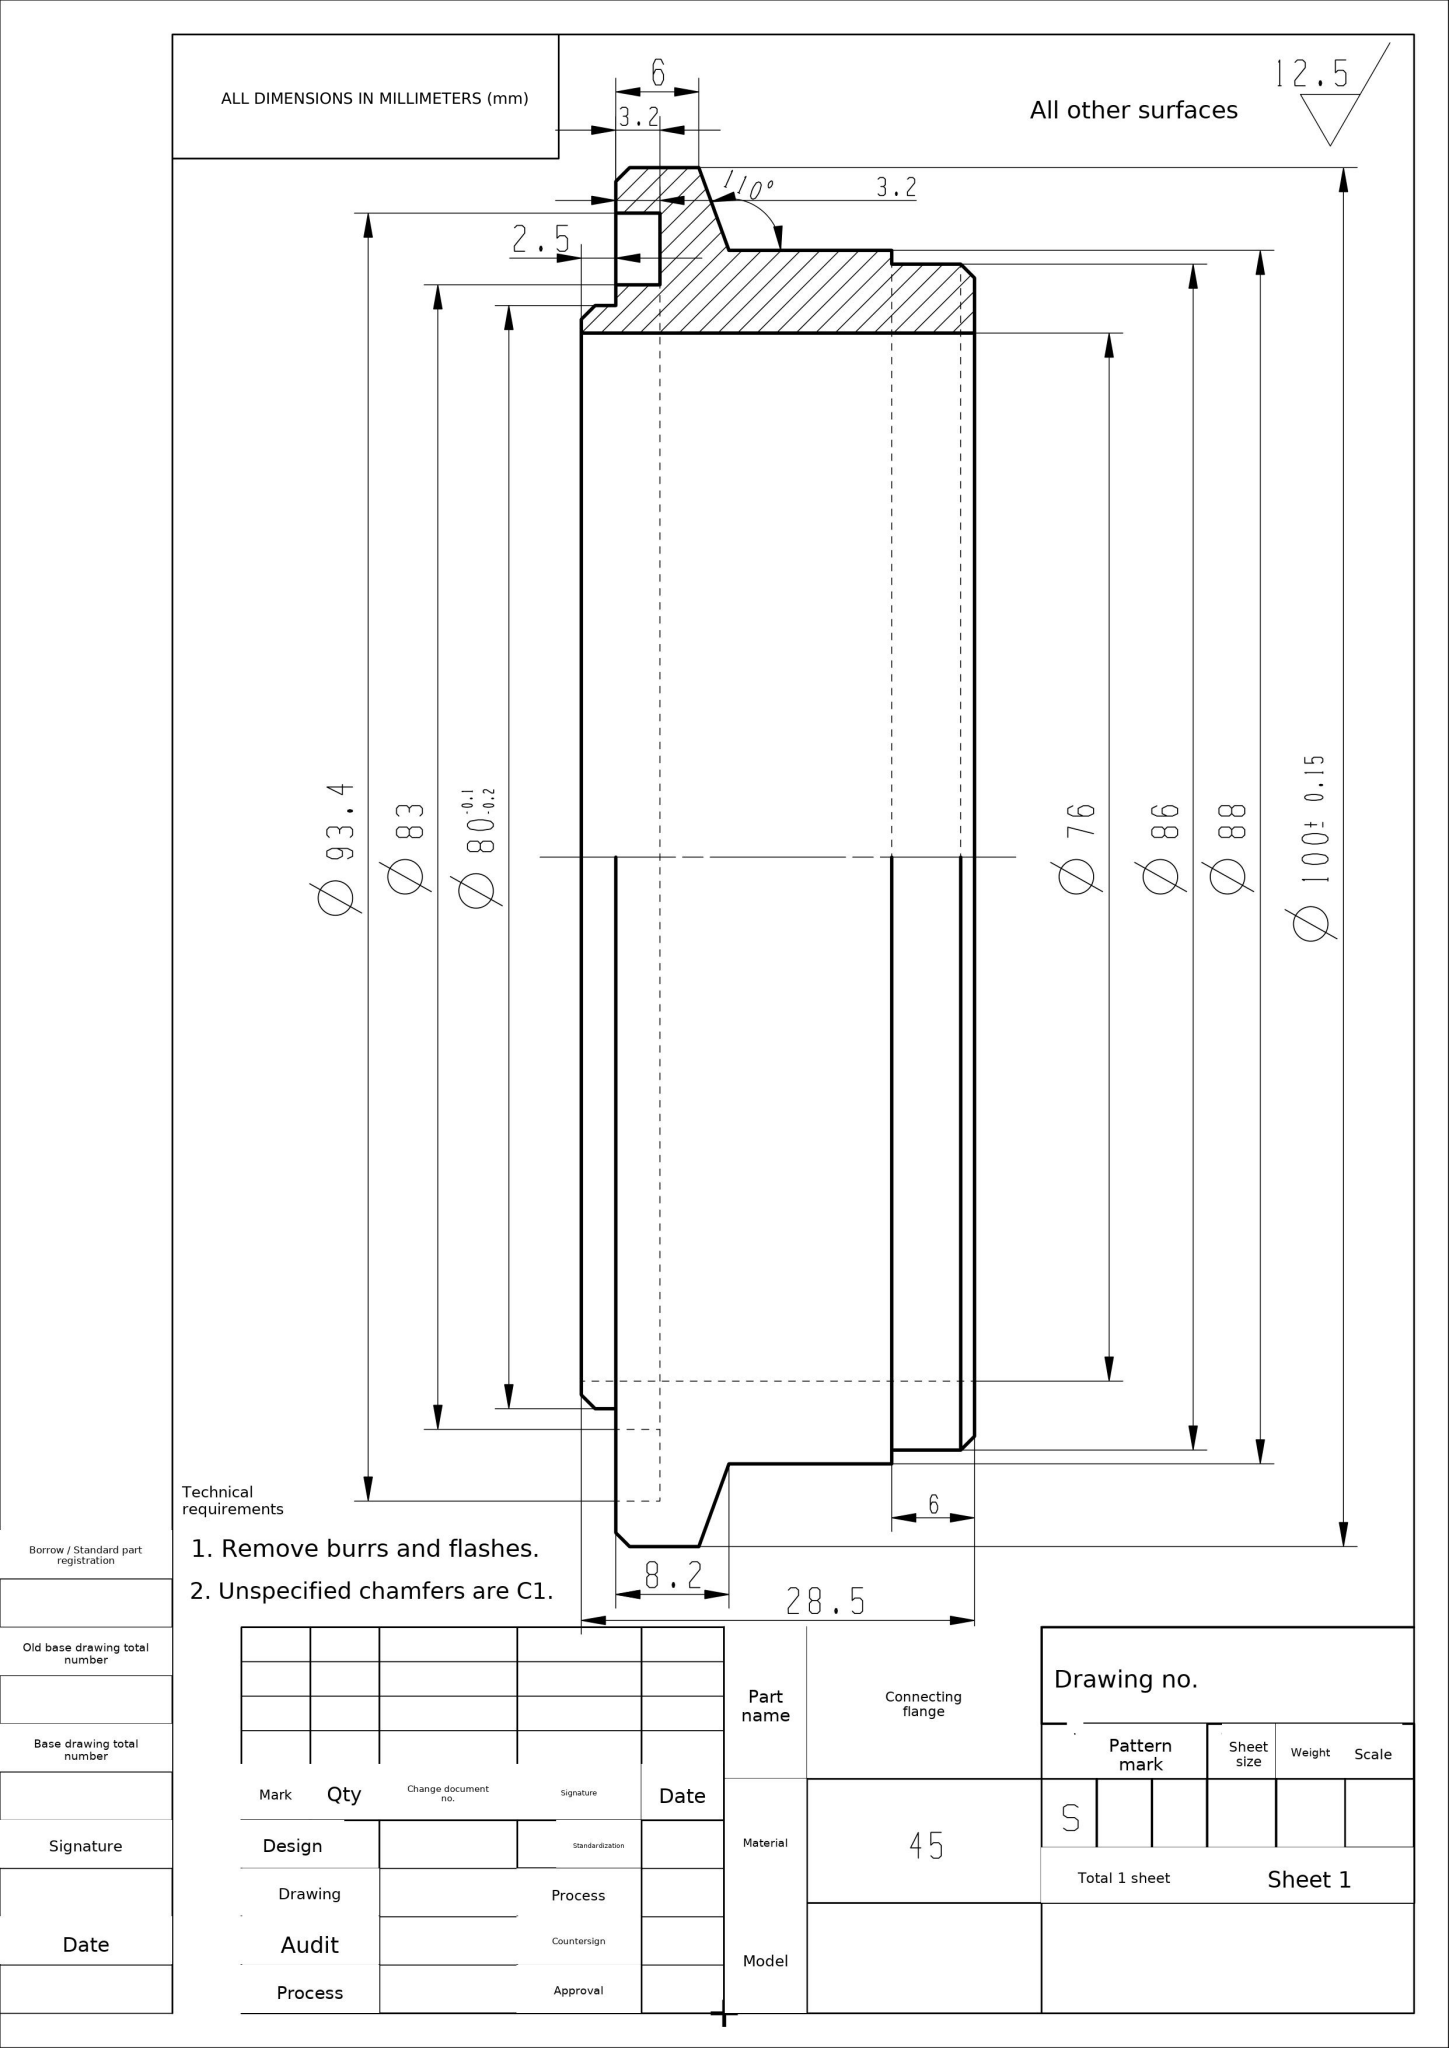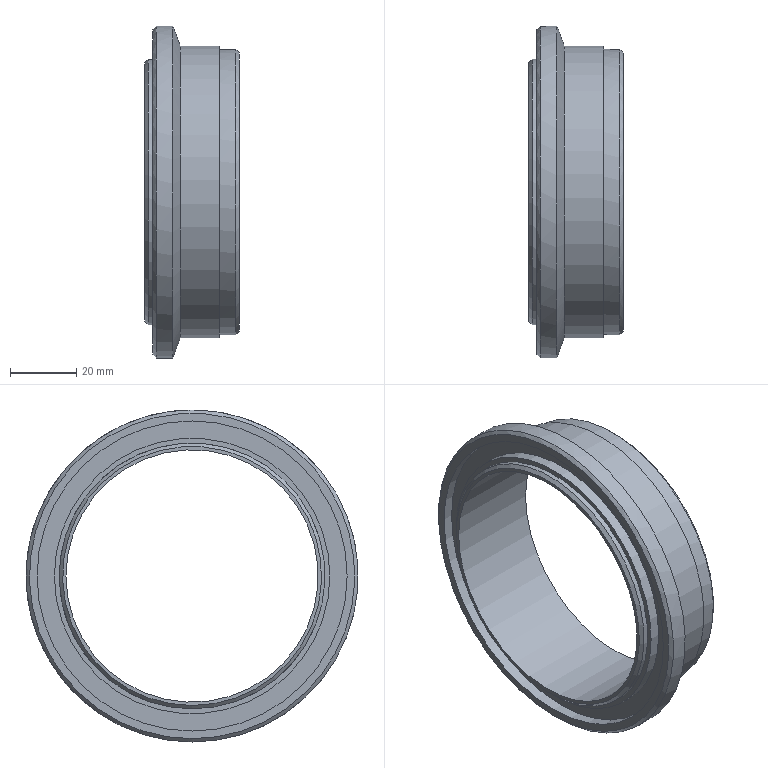Part | NX | mm | 1 solid | 17 faces | box 28.5 x 100 x 100 mm | volume 47300 mm3 | cylinder 7 | plane 6 | cone 4 | commonest cylinder face diameters 88 x1 100 x1 76 x1 80 x1 86 x1 93.4 x1 83 x1
STEP:
#1=CARTESIAN_POINT('',(0.,0.,0.));
#2=DIRECTION('',(0.,0.,1.));
#3=DIRECTION('',(1.,0.,0.));
#4=AXIS2_PLACEMENT_3D('',#1,#2,#3);
#5=(LENGTH_UNIT()NAMED_UNIT(*)SI_UNIT(.MILLI.,.METRE.));
#6=UNCERTAINTY_MEASURE_WITH_UNIT(LENGTH_MEASURE(0.00002),#5,'','');
#7=(NAMED_UNIT(*)PLANE_ANGLE_UNIT()SI_UNIT($,.RADIAN.));
#8=PLANE_ANGLE_MEASURE_WITH_UNIT(PLANE_ANGLE_MEASURE(0.01745),#7);
#9=DIMENSIONAL_EXPONENTS(0.,0.,0.,0.,0.,0.,0.);
#10=(CONVERSION_BASED_UNIT('',#8)NAMED_UNIT(#9)PLANE_ANGLE_UNIT());
#11=(NAMED_UNIT(*)SI_UNIT($,.STERADIAN.)SOLID_ANGLE_UNIT());
#12=(GEOMETRIC_REPRESENTATION_CONTEXT(3)GLOBAL_UNCERTAINTY_ASSIGNED_CONTEXT((#6))GLOBAL_UNIT_ASSIGNED_CONTEXT((#5,#10,#11))REPRESENTATION_CONTEXT('',''));
#13=SHAPE_REPRESENTATION('',(#4),#12);
#14=CARTESIAN_POINT('',(0.,40.,-0.));
#15=VERTEX_POINT('',#14);
#16=CARTESIAN_POINT('',(0.,0.,0.));
#17=DIRECTION('',(1.,0.,0.));
#18=DIRECTION('',(0.,1.,-0.));
#19=AXIS2_PLACEMENT_3D('',#16,#17,#18);
#20=CIRCLE('',#19,40.);
#21=EDGE_CURVE('',#15,#15,#20,.T.);
#22=ORIENTED_EDGE('',*,*,#21,.T.);
#23=EDGE_LOOP('',(#22));
#24=FACE_BOUND('',#23,.T.);
#25=CARTESIAN_POINT('',(0.,41.5,0.));
#26=VERTEX_POINT('',#25);
#27=CARTESIAN_POINT('',(0.,0.,0.));
#28=DIRECTION('',(-1.,0.,0.));
#29=DIRECTION('',(0.,1.,0.));
#30=AXIS2_PLACEMENT_3D('',#27,#28,#29);
#31=CIRCLE('',#30,41.5);
#32=EDGE_CURVE('',#26,#26,#31,.T.);
#33=ORIENTED_EDGE('',*,*,#32,.T.);
#34=EDGE_LOOP('',(#33));
#35=FACE_BOUND('',#34,.T.);
#36=CARTESIAN_POINT('',(0.,0.,0.));
#37=DIRECTION('',(1.,0.,0.));
#38=DIRECTION('',(0.,0.,-1.));
#39=AXIS2_PLACEMENT_3D('',#36,#37,#38);
#40=PLANE('',#39);
#41=ADVANCED_FACE('',(#24,#35),#40,.F.);
#42=CARTESIAN_POINT('',(8.2,44.,-0.));
#43=VERTEX_POINT('',#42);
#44=CARTESIAN_POINT('',(8.2,0.,0.));
#45=DIRECTION('',(1.,0.,0.));
#46=DIRECTION('',(0.,1.,-0.));
#47=AXIS2_PLACEMENT_3D('',#44,#45,#46);
#48=CIRCLE('',#47,44.);
#49=EDGE_CURVE('',#43,#43,#48,.T.);
#50=ORIENTED_EDGE('',*,*,#49,.T.);
#51=EDGE_LOOP('',(#50));
#52=FACE_BOUND('',#51,.T.);
#53=CARTESIAN_POINT('',(20.,44.,-0.));
#54=VERTEX_POINT('',#53);
#55=CARTESIAN_POINT('',(20.,0.,0.));
#56=DIRECTION('',(1.,0.,0.));
#57=DIRECTION('',(0.,1.,-0.));
#58=AXIS2_PLACEMENT_3D('',#55,#56,#57);
#59=CIRCLE('',#58,44.);
#60=EDGE_CURVE('',#54,#54,#59,.T.);
#61=ORIENTED_EDGE('',*,*,#60,.F.);
#62=EDGE_LOOP('',(#61));
#63=FACE_BOUND('',#62,.T.);
#64=CARTESIAN_POINT('',(26.,0.,0.));
#65=DIRECTION('',(-1.,0.,0.));
#66=DIRECTION('',(0.,0.,1.));
#67=AXIS2_PLACEMENT_3D('',#64,#65,#66);
#68=CYLINDRICAL_SURFACE('',#67,44.);
#69=ADVANCED_FACE('',(#52,#63),#68,.T.);
#70=CARTESIAN_POINT('',(26.,0.,-42.));
#71=VERTEX_POINT('',#70);
#72=CARTESIAN_POINT('',(26.,0.,0.));
#73=DIRECTION('',(1.,0.,0.));
#74=DIRECTION('',(0.,0.,-1.));
#75=AXIS2_PLACEMENT_3D('',#72,#73,#74);
#76=CIRCLE('',#75,42.);
#77=EDGE_CURVE('',#71,#71,#76,.T.);
#78=ORIENTED_EDGE('',*,*,#77,.T.);
#79=EDGE_LOOP('',(#78));
#80=FACE_BOUND('',#79,.T.);
#81=CARTESIAN_POINT('',(26.,38.,-0.));
#82=VERTEX_POINT('',#81);
#83=CARTESIAN_POINT('',(26.,0.,0.));
#84=DIRECTION('',(1.,0.,0.));
#85=DIRECTION('',(0.,1.,-0.));
#86=AXIS2_PLACEMENT_3D('',#83,#84,#85);
#87=CIRCLE('',#86,38.);
#88=EDGE_CURVE('',#82,#82,#87,.T.);
#89=ORIENTED_EDGE('',*,*,#88,.F.);
#90=EDGE_LOOP('',(#89));
#91=FACE_BOUND('',#90,.T.);
#92=CARTESIAN_POINT('',(26.,0.,0.));
#93=DIRECTION('',(1.,0.,0.));
#94=DIRECTION('',(0.,0.,-1.));
#95=AXIS2_PLACEMENT_3D('',#92,#93,#94);
#96=PLANE('',#95);
#97=ADVANCED_FACE('',(#80,#91),#96,.T.);
#98=CARTESIAN_POINT('',(1.,0.,-50.));
#99=VERTEX_POINT('',#98);
#100=CARTESIAN_POINT('',(1.,0.,0.));
#101=DIRECTION('',(1.,0.,0.));
#102=DIRECTION('',(0.,0.,-1.));
#103=AXIS2_PLACEMENT_3D('',#100,#101,#102);
#104=CIRCLE('',#103,50.);
#105=EDGE_CURVE('',#99,#99,#104,.T.);
#106=ORIENTED_EDGE('',*,*,#105,.T.);
#107=EDGE_LOOP('',(#106));
#108=FACE_BOUND('',#107,.T.);
#109=CARTESIAN_POINT('',(6.016,0.,-50.));
#110=VERTEX_POINT('',#109);
#111=CARTESIAN_POINT('',(6.016,0.,0.));
#112=DIRECTION('',(-1.,0.,0.));
#113=DIRECTION('',(0.,0.,-1.));
#114=AXIS2_PLACEMENT_3D('',#111,#112,#113);
#115=CIRCLE('',#114,50.);
#116=EDGE_CURVE('',#110,#110,#115,.T.);
#117=ORIENTED_EDGE('',*,*,#116,.T.);
#118=EDGE_LOOP('',(#117));
#119=FACE_BOUND('',#118,.T.);
#120=CARTESIAN_POINT('',(8.2,0.,0.));
#121=DIRECTION('',(-1.,0.,0.));
#122=DIRECTION('',(0.,0.,1.));
#123=AXIS2_PLACEMENT_3D('',#120,#121,#122);
#124=CYLINDRICAL_SURFACE('',#123,50.);
#125=ADVANCED_FACE('',(#108,#119),#124,.T.);
#126=CARTESIAN_POINT('',(-2.5,38.,-0.));
#127=VERTEX_POINT('',#126);
#128=CARTESIAN_POINT('',(-2.5,0.,0.));
#129=DIRECTION('',(1.,0.,0.));
#130=DIRECTION('',(0.,1.,-0.));
#131=AXIS2_PLACEMENT_3D('',#128,#129,#130);
#132=CIRCLE('',#131,38.);
#133=EDGE_CURVE('',#127,#127,#132,.T.);
#134=ORIENTED_EDGE('',*,*,#133,.F.);
#135=EDGE_LOOP('',(#134));
#136=FACE_BOUND('',#135,.T.);
#137=ORIENTED_EDGE('',*,*,#88,.T.);
#138=EDGE_LOOP('',(#137));
#139=FACE_BOUND('',#138,.T.);
#140=CARTESIAN_POINT('',(8.2,0.,0.));
#141=DIRECTION('',(-1.,0.,0.));
#142=DIRECTION('',(0.,0.,1.));
#143=AXIS2_PLACEMENT_3D('',#140,#141,#142);
#144=CYLINDRICAL_SURFACE('',#143,38.);
#145=ADVANCED_FACE('',(#136,#139),#144,.F.);
#146=CARTESIAN_POINT('',(0.,46.7,0.));
#147=VERTEX_POINT('',#146);
#148=CARTESIAN_POINT('',(0.,0.,0.));
#149=DIRECTION('',(-1.,0.,0.));
#150=DIRECTION('',(0.,1.,0.));
#151=AXIS2_PLACEMENT_3D('',#148,#149,#150);
#152=CIRCLE('',#151,46.7);
#153=EDGE_CURVE('',#147,#147,#152,.T.);
#154=ORIENTED_EDGE('',*,*,#153,.F.);
#155=EDGE_LOOP('',(#154));
#156=FACE_BOUND('',#155,.T.);
#157=CARTESIAN_POINT('',(0.,0.,-49.));
#158=VERTEX_POINT('',#157);
#159=CARTESIAN_POINT('',(0.,0.,0.));
#160=DIRECTION('',(-1.,0.,0.));
#161=DIRECTION('',(0.,0.,-1.));
#162=AXIS2_PLACEMENT_3D('',#159,#160,#161);
#163=CIRCLE('',#162,49.);
#164=EDGE_CURVE('',#158,#158,#163,.T.);
#165=ORIENTED_EDGE('',*,*,#164,.T.);
#166=EDGE_LOOP('',(#165));
#167=FACE_BOUND('',#166,.T.);
#168=CARTESIAN_POINT('',(0.,0.,0.));
#169=DIRECTION('',(1.,0.,0.));
#170=DIRECTION('',(0.,0.,-1.));
#171=AXIS2_PLACEMENT_3D('',#168,#169,#170);
#172=PLANE('',#171);
#173=ADVANCED_FACE('',(#156,#167),#172,.F.);
#174=CARTESIAN_POINT('',(-1.5,0.,-40.));
#175=VERTEX_POINT('',#174);
#176=CARTESIAN_POINT('',(-1.5,0.,0.));
#177=DIRECTION('',(1.,0.,0.));
#178=DIRECTION('',(0.,0.,-1.));
#179=AXIS2_PLACEMENT_3D('',#176,#177,#178);
#180=CIRCLE('',#179,40.);
#181=EDGE_CURVE('',#175,#175,#180,.T.);
#182=ORIENTED_EDGE('',*,*,#181,.T.);
#183=EDGE_LOOP('',(#182));
#184=FACE_BOUND('',#183,.T.);
#185=ORIENTED_EDGE('',*,*,#21,.F.);
#186=EDGE_LOOP('',(#185));
#187=FACE_BOUND('',#186,.T.);
#188=CARTESIAN_POINT('',(-2.5,0.,0.));
#189=DIRECTION('',(1.,0.,0.));
#190=DIRECTION('',(0.,0.,-1.));
#191=AXIS2_PLACEMENT_3D('',#188,#189,#190);
#192=CYLINDRICAL_SURFACE('',#191,40.);
#193=ADVANCED_FACE('',(#184,#187),#192,.T.);
#194=CARTESIAN_POINT('',(-2.5,0.,-39.));
#195=VERTEX_POINT('',#194);
#196=CARTESIAN_POINT('',(-2.5,0.,0.));
#197=DIRECTION('',(-1.,0.,0.));
#198=DIRECTION('',(0.,0.,-1.));
#199=AXIS2_PLACEMENT_3D('',#196,#197,#198);
#200=CIRCLE('',#199,39.);
#201=EDGE_CURVE('',#195,#195,#200,.T.);
#202=ORIENTED_EDGE('',*,*,#201,.T.);
#203=EDGE_LOOP('',(#202));
#204=FACE_BOUND('',#203,.T.);
#205=ORIENTED_EDGE('',*,*,#133,.T.);
#206=EDGE_LOOP('',(#205));
#207=FACE_BOUND('',#206,.T.);
#208=CARTESIAN_POINT('',(-2.5,0.,0.));
#209=DIRECTION('',(1.,0.,0.));
#210=DIRECTION('',(0.,0.,-1.));
#211=AXIS2_PLACEMENT_3D('',#208,#209,#210);
#212=PLANE('',#211);
#213=ADVANCED_FACE('',(#204,#207),#212,.F.);
#214=CARTESIAN_POINT('',(25.,0.,-43.));
#215=VERTEX_POINT('',#214);
#216=CARTESIAN_POINT('',(25.,0.,0.));
#217=DIRECTION('',(-1.,0.,0.));
#218=DIRECTION('',(0.,0.,-1.));
#219=AXIS2_PLACEMENT_3D('',#216,#217,#218);
#220=CIRCLE('',#219,43.);
#221=EDGE_CURVE('',#215,#215,#220,.T.);
#222=ORIENTED_EDGE('',*,*,#221,.T.);
#223=EDGE_LOOP('',(#222));
#224=FACE_BOUND('',#223,.T.);
#225=CARTESIAN_POINT('',(20.,43.,-0.));
#226=VERTEX_POINT('',#225);
#227=CARTESIAN_POINT('',(20.,0.,0.));
#228=DIRECTION('',(-1.,0.,0.));
#229=DIRECTION('',(0.,1.,-0.));
#230=AXIS2_PLACEMENT_3D('',#227,#228,#229);
#231=CIRCLE('',#230,43.);
#232=EDGE_CURVE('',#226,#226,#231,.T.);
#233=ORIENTED_EDGE('',*,*,#232,.F.);
#234=EDGE_LOOP('',(#233));
#235=FACE_BOUND('',#234,.T.);
#236=CARTESIAN_POINT('',(20.,0.,0.));
#237=DIRECTION('',(1.,0.,0.));
#238=DIRECTION('',(0.,0.,-1.));
#239=AXIS2_PLACEMENT_3D('',#236,#237,#238);
#240=CYLINDRICAL_SURFACE('',#239,43.);
#241=ADVANCED_FACE('',(#224,#235),#240,.T.);
#242=ORIENTED_EDGE('',*,*,#60,.T.);
#243=EDGE_LOOP('',(#242));
#244=FACE_BOUND('',#243,.T.);
#245=ORIENTED_EDGE('',*,*,#232,.T.);
#246=EDGE_LOOP('',(#245));
#247=FACE_BOUND('',#246,.T.);
#248=CARTESIAN_POINT('',(20.,0.,0.));
#249=DIRECTION('',(1.,0.,0.));
#250=DIRECTION('',(0.,0.,-1.));
#251=AXIS2_PLACEMENT_3D('',#248,#249,#250);
#252=PLANE('',#251);
#253=ADVANCED_FACE('',(#244,#247),#252,.T.);
#254=ORIENTED_EDGE('',*,*,#116,.F.);
#255=EDGE_LOOP('',(#254));
#256=FACE_BOUND('',#255,.T.);
#257=ORIENTED_EDGE('',*,*,#49,.F.);
#258=EDGE_LOOP('',(#257));
#259=FACE_BOUND('',#258,.T.);
#260=CARTESIAN_POINT('',(8.2,0.,0.));
#261=DIRECTION('',(-1.,0.,0.));
#262=DIRECTION('',(-0.,0.,1.));
#263=AXIS2_PLACEMENT_3D('',#260,#261,#262);
#264=CONICAL_SURFACE('',#263,44.,70.);
#265=ADVANCED_FACE('',(#256,#259),#264,.T.);
#266=ORIENTED_EDGE('',*,*,#164,.F.);
#267=EDGE_LOOP('',(#266));
#268=FACE_BOUND('',#267,.T.);
#269=ORIENTED_EDGE('',*,*,#105,.F.);
#270=EDGE_LOOP('',(#269));
#271=FACE_BOUND('',#270,.T.);
#272=CARTESIAN_POINT('',(1.,0.,0.));
#273=DIRECTION('',(1.,0.,0.));
#274=DIRECTION('',(-0.,0.,-1.));
#275=AXIS2_PLACEMENT_3D('',#272,#273,#274);
#276=CONICAL_SURFACE('',#275,50.,45.);
#277=ADVANCED_FACE('',(#268,#271),#276,.T.);
#278=ORIENTED_EDGE('',*,*,#201,.F.);
#279=EDGE_LOOP('',(#278));
#280=FACE_BOUND('',#279,.T.);
#281=ORIENTED_EDGE('',*,*,#181,.F.);
#282=EDGE_LOOP('',(#281));
#283=FACE_BOUND('',#282,.T.);
#284=CARTESIAN_POINT('',(-1.5,0.,0.));
#285=DIRECTION('',(1.,0.,0.));
#286=DIRECTION('',(0.,0.,-1.));
#287=AXIS2_PLACEMENT_3D('',#284,#285,#286);
#288=CONICAL_SURFACE('',#287,40.,45.);
#289=ADVANCED_FACE('',(#280,#283),#288,.T.);
#290=CARTESIAN_POINT('',(3.2,46.7,0.));
#291=VERTEX_POINT('',#290);
#292=CARTESIAN_POINT('',(3.2,0.,0.));
#293=DIRECTION('',(1.,0.,0.));
#294=DIRECTION('',(0.,1.,0.));
#295=AXIS2_PLACEMENT_3D('',#292,#293,#294);
#296=CIRCLE('',#295,46.7);
#297=EDGE_CURVE('',#291,#291,#296,.T.);
#298=ORIENTED_EDGE('',*,*,#297,.T.);
#299=EDGE_LOOP('',(#298));
#300=FACE_BOUND('',#299,.T.);
#301=ORIENTED_EDGE('',*,*,#153,.T.);
#302=EDGE_LOOP('',(#301));
#303=FACE_BOUND('',#302,.T.);
#304=CARTESIAN_POINT('',(3.2,0.,0.));
#305=DIRECTION('',(-1.,0.,0.));
#306=DIRECTION('',(0.,0.,1.));
#307=AXIS2_PLACEMENT_3D('',#304,#305,#306);
#308=CYLINDRICAL_SURFACE('',#307,46.7);
#309=ADVANCED_FACE('',(#300,#303),#308,.F.);
#310=CARTESIAN_POINT('',(3.2,41.5,0.));
#311=VERTEX_POINT('',#310);
#312=CARTESIAN_POINT('',(3.2,0.,0.));
#313=DIRECTION('',(1.,0.,0.));
#314=DIRECTION('',(0.,1.,0.));
#315=AXIS2_PLACEMENT_3D('',#312,#313,#314);
#316=CIRCLE('',#315,41.5);
#317=EDGE_CURVE('',#311,#311,#316,.T.);
#318=ORIENTED_EDGE('',*,*,#317,.F.);
#319=EDGE_LOOP('',(#318));
#320=FACE_BOUND('',#319,.T.);
#321=ORIENTED_EDGE('',*,*,#32,.F.);
#322=EDGE_LOOP('',(#321));
#323=FACE_BOUND('',#322,.T.);
#324=CARTESIAN_POINT('',(3.2,0.,0.));
#325=DIRECTION('',(-1.,0.,0.));
#326=DIRECTION('',(0.,0.,1.));
#327=AXIS2_PLACEMENT_3D('',#324,#325,#326);
#328=CYLINDRICAL_SURFACE('',#327,41.5);
#329=ADVANCED_FACE('',(#320,#323),#328,.T.);
#330=ORIENTED_EDGE('',*,*,#297,.F.);
#331=EDGE_LOOP('',(#330));
#332=FACE_BOUND('',#331,.T.);
#333=ORIENTED_EDGE('',*,*,#317,.T.);
#334=EDGE_LOOP('',(#333));
#335=FACE_BOUND('',#334,.T.);
#336=CARTESIAN_POINT('',(3.2,0.,0.));
#337=DIRECTION('',(-1.,0.,0.));
#338=DIRECTION('',(0.,0.,1.));
#339=AXIS2_PLACEMENT_3D('',#336,#337,#338);
#340=PLANE('',#339);
#341=ADVANCED_FACE('',(#332,#335),#340,.T.);
#342=ORIENTED_EDGE('',*,*,#221,.F.);
#343=EDGE_LOOP('',(#342));
#344=FACE_BOUND('',#343,.T.);
#345=ORIENTED_EDGE('',*,*,#77,.F.);
#346=EDGE_LOOP('',(#345));
#347=FACE_BOUND('',#346,.T.);
#348=CARTESIAN_POINT('',(26.,0.,0.));
#349=DIRECTION('',(-1.,0.,0.));
#350=DIRECTION('',(0.,0.,1.));
#351=AXIS2_PLACEMENT_3D('',#348,#349,#350);
#352=CONICAL_SURFACE('',#351,42.,45.);
#353=ADVANCED_FACE('',(#344,#347),#352,.T.);
#354=CLOSED_SHELL('',(#41,#69,#97,#125,#145,#173,#193,#213,#241,#253,#265,#277,#289,#309,#329,#341,#353));
#355=MANIFOLD_SOLID_BREP('',#354);
#356=ADVANCED_BREP_SHAPE_REPRESENTATION('',(#355),#12);
#357=SHAPE_REPRESENTATION_RELATIONSHIP('','',#13,#356);
#358=PRESENTATION_LAYER_ASSIGNMENT('','',(#355));
#359=COLOUR_RGB('',1.,0.6,0.);
#360=FILL_AREA_STYLE_COLOUR('',#359);
#361=FILL_AREA_STYLE('',(#360));
#362=SURFACE_STYLE_FILL_AREA(#361);
#363=SURFACE_SIDE_STYLE('',(#362));
#364=SURFACE_STYLE_USAGE(.BOTH.,#363);
#365=PRESENTATION_STYLE_ASSIGNMENT((#364));
#366=STYLED_ITEM('',(#365),#355);
#367=MECHANICAL_DESIGN_GEOMETRIC_PRESENTATION_REPRESENTATION('',(#366),#12);